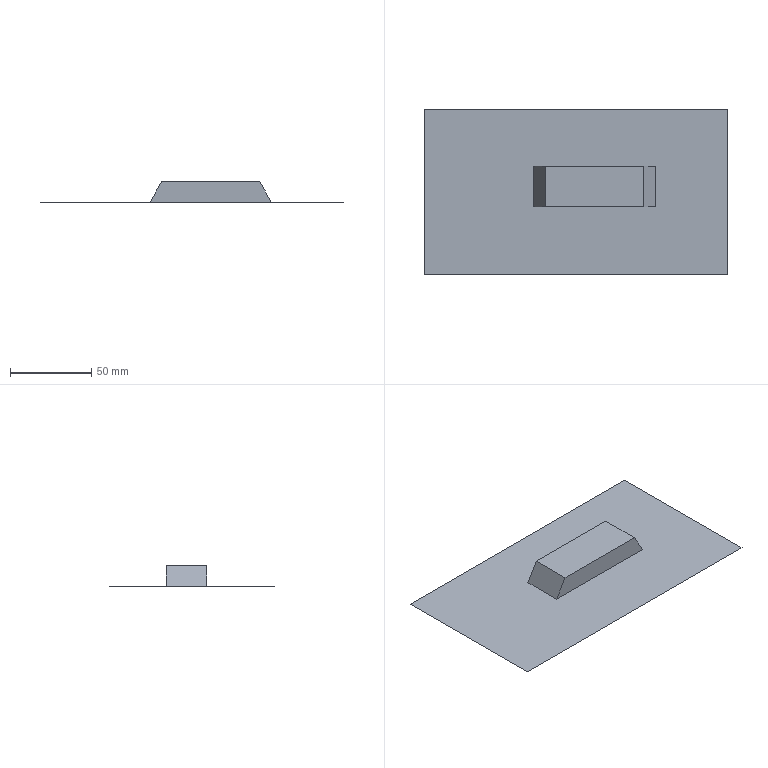CAM job | Mastercam | mm | 2 operations | part box 186.94 x 101.95 x 12.6
1. Surface Finish Flowline | 2 - 12 平铣刀
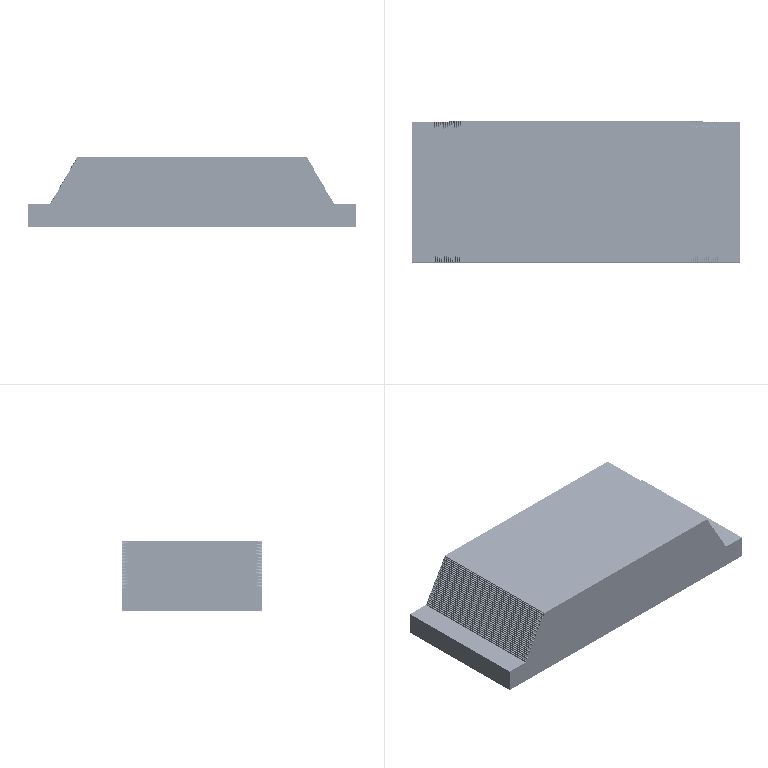2. Surface Finish Flowline | 24 - 10 圆鼻铣刀